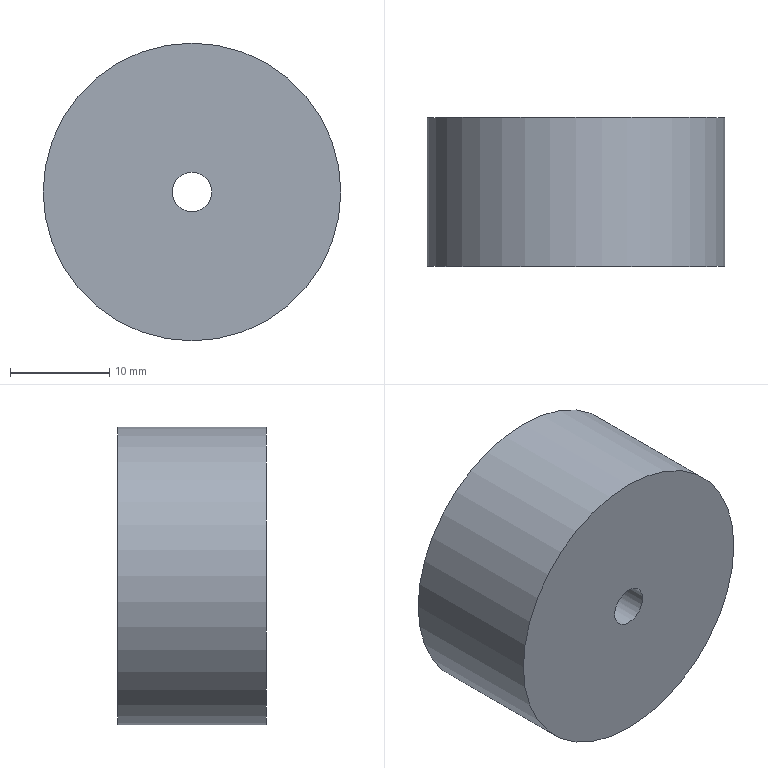Component | NX | REAR_WHEEL | 1 solid | 24 faces | volume 8639 mm3 | cylinder 8 | sphere 6 | torus 6 | plane 3 | cone 1 | commonest cylinder face diameters 8 x6 30 x1 4 x1